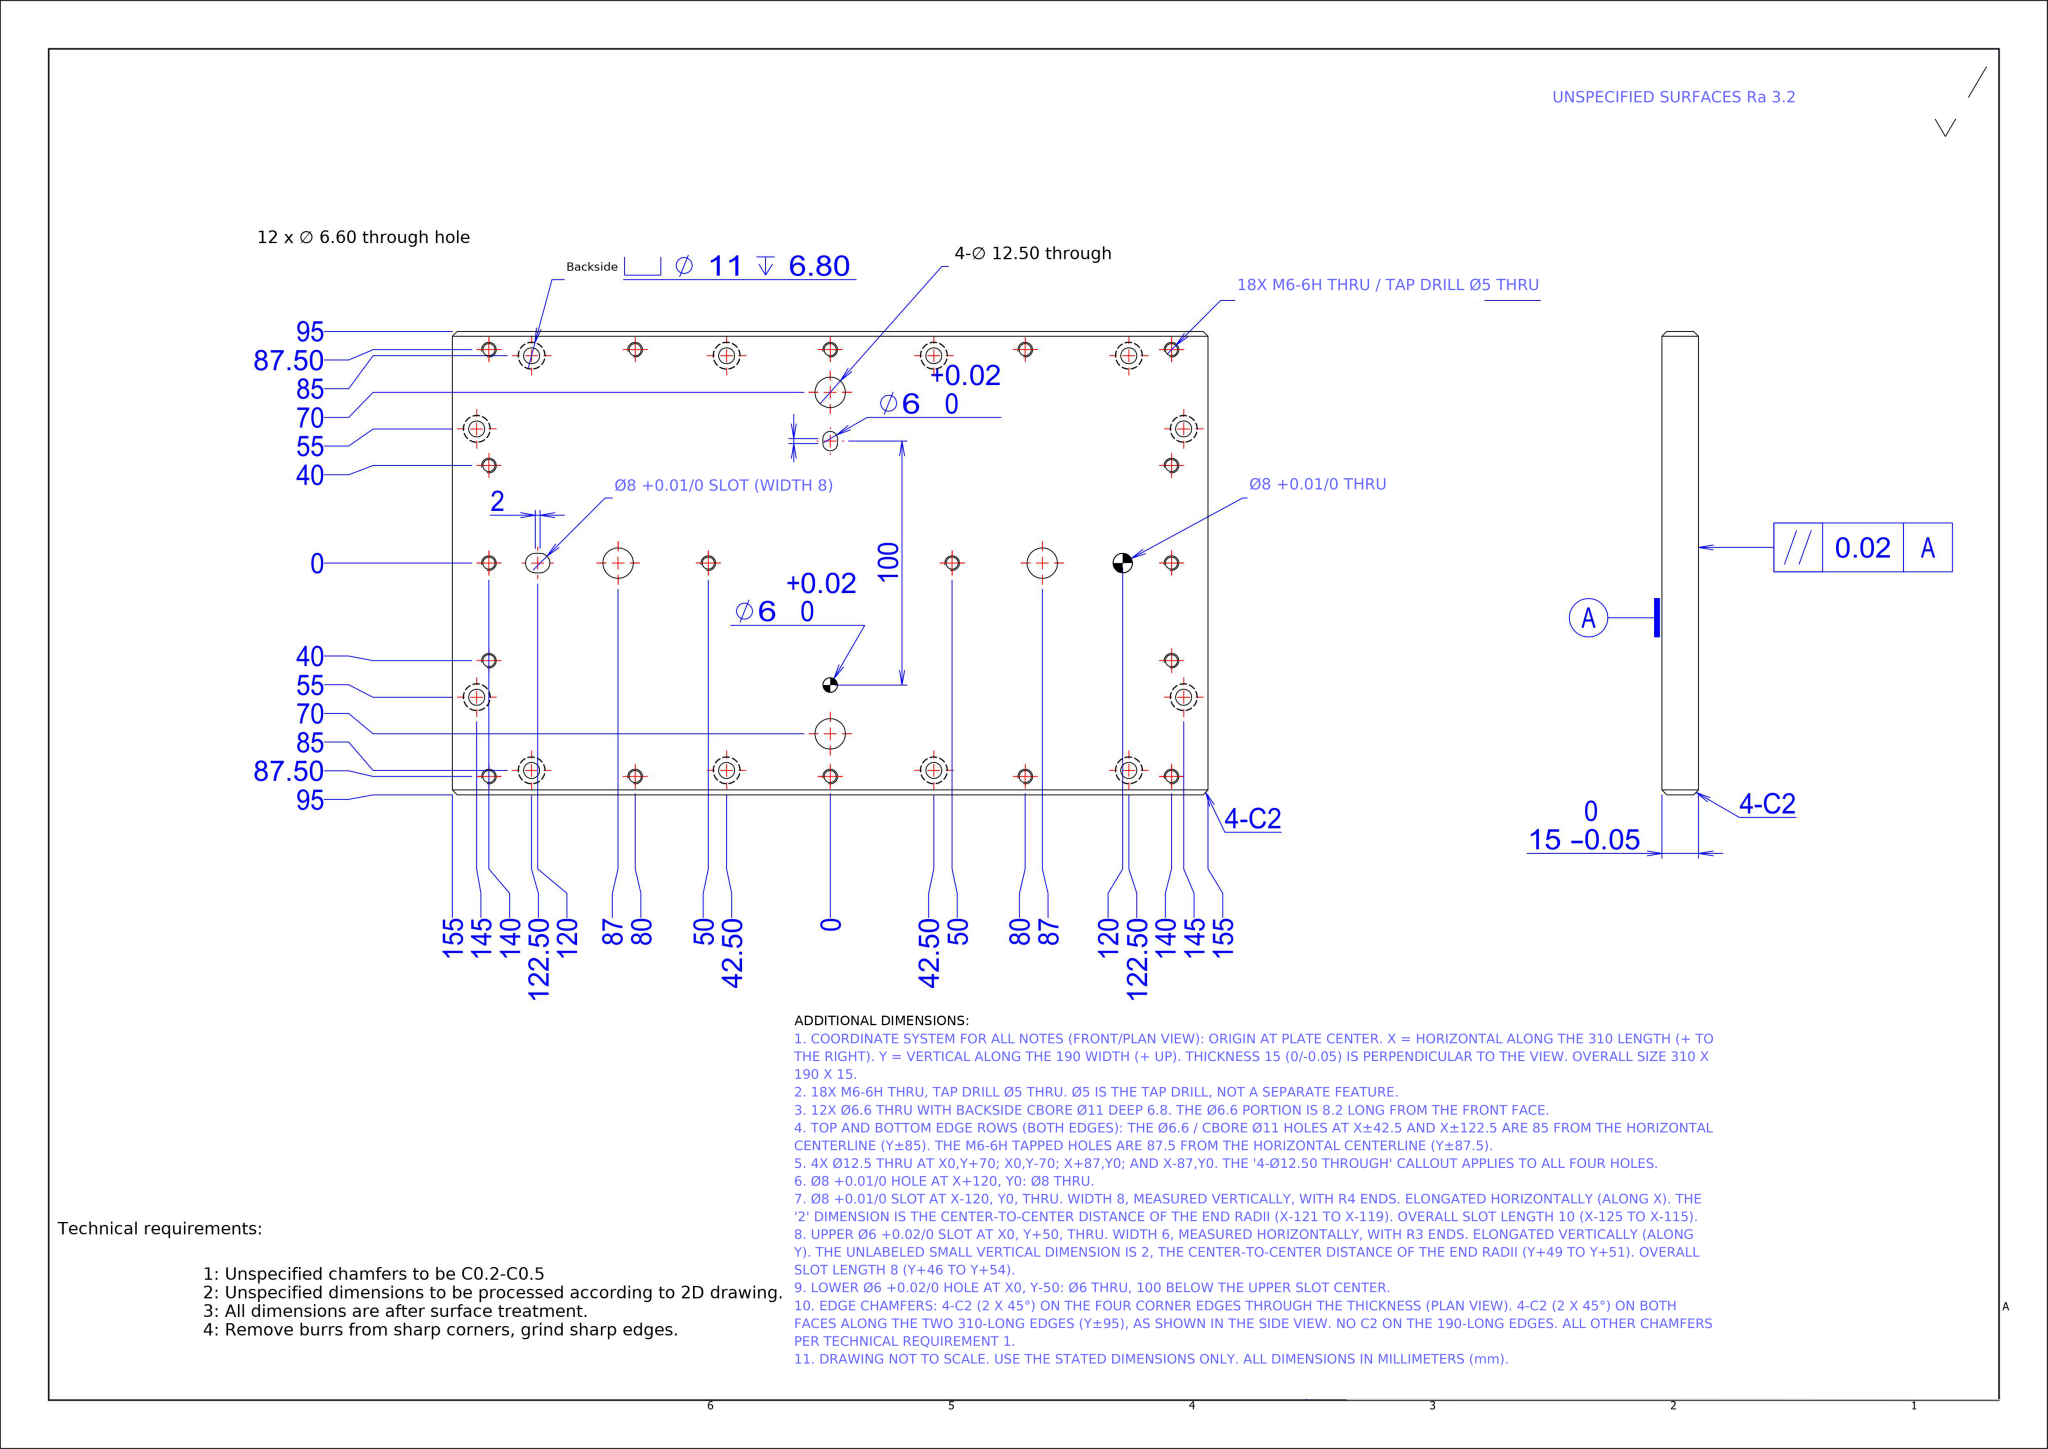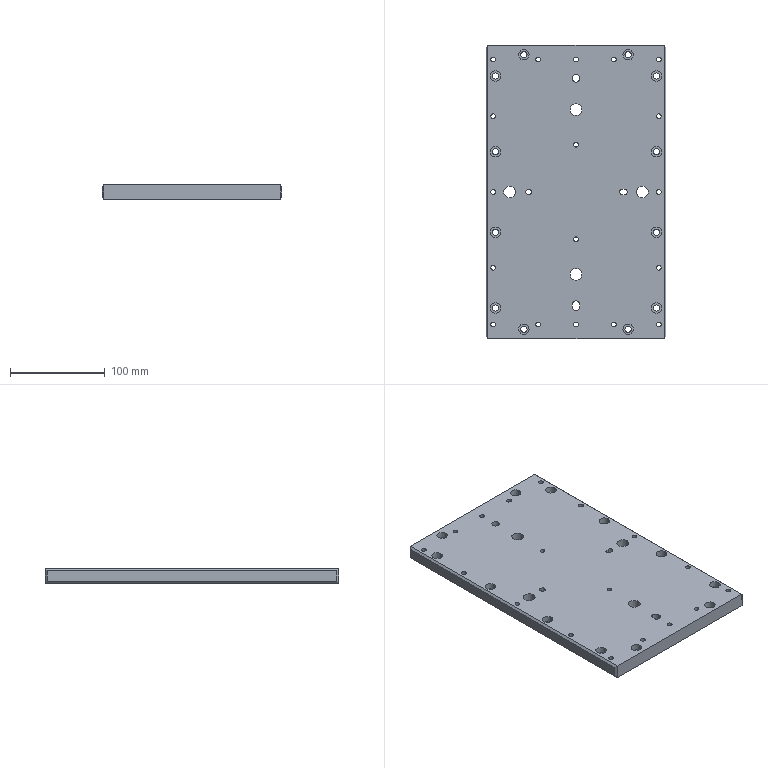Part | NX | mm | 1 solid | 131 faces | box 190 x 310 x 15 mm | volume 854359 mm3 | cylinder 101 | plane 30 | commonest cylinder face diameters 5 x36 11 x24 6.6 x24 12.5 x8 6 x5 8 x4